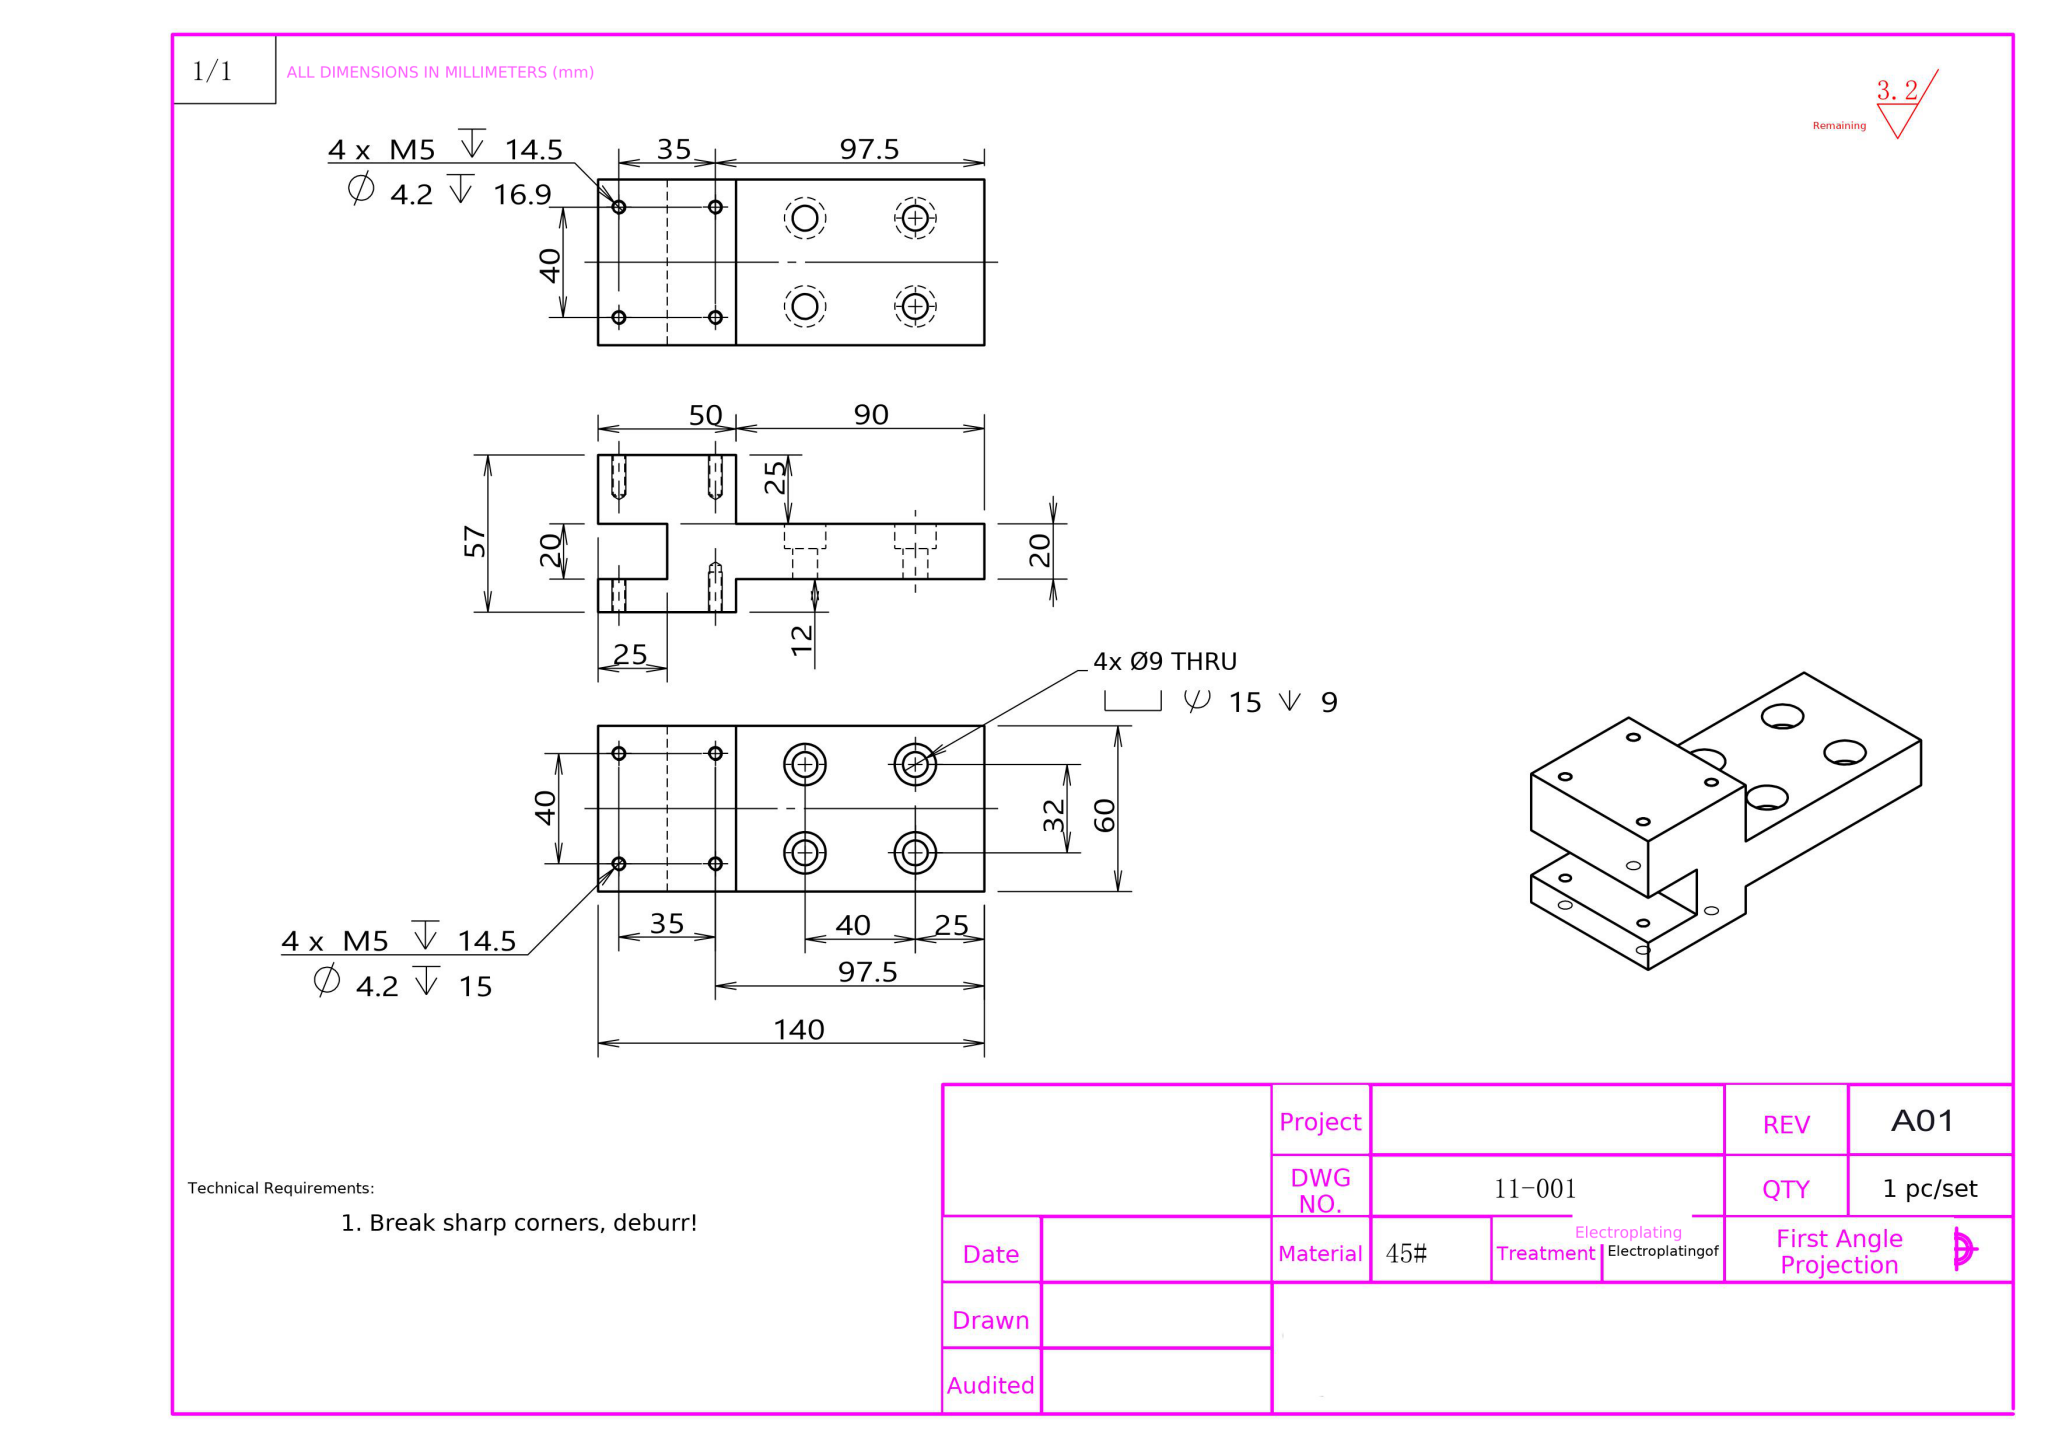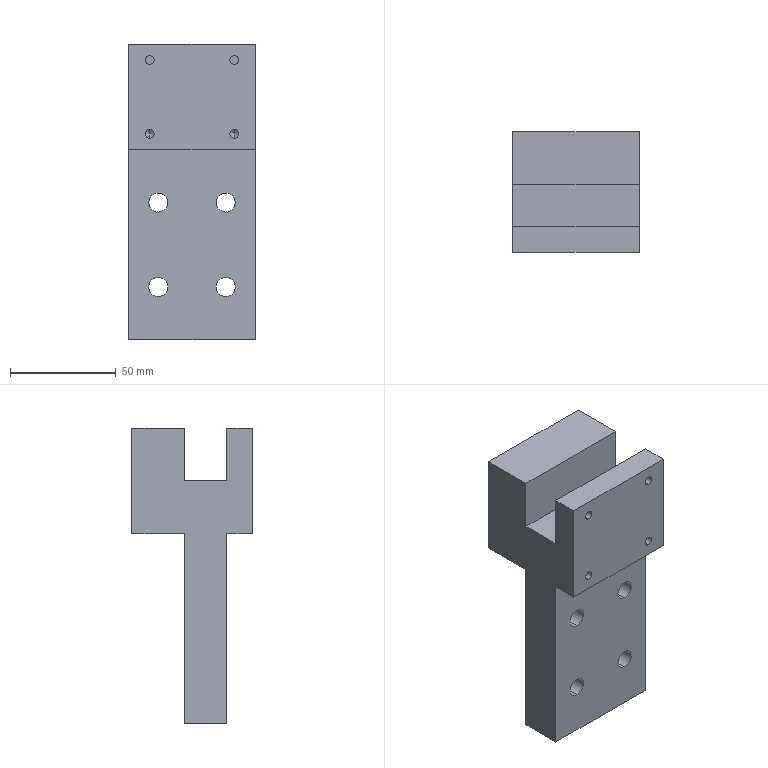Part | NX | mm | 1 solid | 62 faces | box 60 x 57 x 140 mm | volume 238172 mm3 | cylinder 32 | plane 18 | cone 12 | commonest cylinder face diameters 4.2 x16 15 x8 9 x8